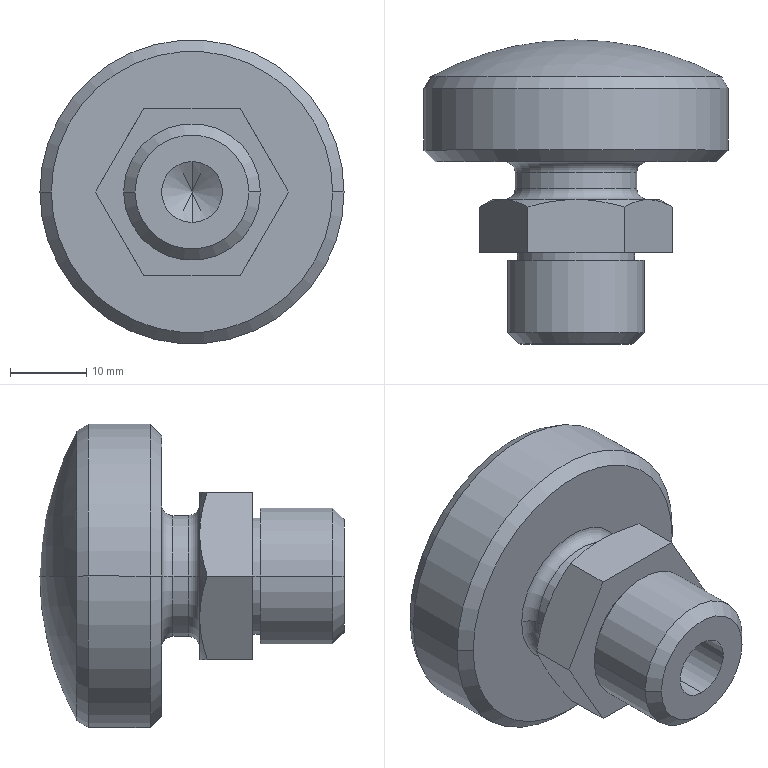Component | SolidWorks | BreatherCap-1 | 1 solid | 37 faces | box 40 x 40 x 40 mm | volume 21828 mm3 | plane 11 | cylinder 10 | cone 10 | torus 4 | sphere 2 | commonest cylinder face diameters 8 x2 15.4 x2 18 x2 16 x2 39.997 x2 | material Q235-A
STEP:
#1=COLOUR_RGB('',0.7922,0.8196,0.9333);
#2=FILL_AREA_STYLE_COLOUR('',#1);
#3=FILL_AREA_STYLE('',(#2));
#4=SURFACE_STYLE_FILL_AREA(#3);
#5=SURFACE_SIDE_STYLE('',(#4));
#6=SURFACE_STYLE_USAGE(.BOTH.,#5);
#7=PRESENTATION_STYLE_ASSIGNMENT((#6));
#8=CARTESIAN_POINT('',(-14.961,3.78,0.1575));
#9=VERTEX_POINT('',#8);
#10=CARTESIAN_POINT('',(-14.961,3.78,-0.1575));
#11=VERTEX_POINT('',#10);
#12=CARTESIAN_POINT('',(-14.961,3.78,0.));
#13=DIRECTION('',(0.,-1.,0.));
#14=DIRECTION('',(0.,0.,-1.));
#15=AXIS2_PLACEMENT_3D('',#12,#13,#14);
#16=CIRCLE('',#15,0.1575);
#17=EDGE_CURVE('',#9,#11,#16,.T.);
#18=ORIENTED_EDGE('',*,*,#17,.F.);
#19=CARTESIAN_POINT('',(-14.961,2.48,0.1575));
#20=VERTEX_POINT('',#19);
#21=CARTESIAN_POINT('',(-14.961,2.48,0.1575));
#22=DIRECTION('',(0.,-1.,0.));
#23=VECTOR('',#22,39.37);
#24=LINE('',#21,#23);
#25=EDGE_CURVE('',#9,#20,#24,.T.);
#26=ORIENTED_EDGE('',*,*,#25,.T.);
#27=CARTESIAN_POINT('',(-14.961,2.48,-0.1575));
#28=VERTEX_POINT('',#27);
#29=CARTESIAN_POINT('',(-14.961,2.48,0.));
#30=DIRECTION('',(0.,-1.,0.));
#31=DIRECTION('',(0.,0.,-1.));
#32=AXIS2_PLACEMENT_3D('',#29,#30,#31);
#33=CIRCLE('',#32,0.1575);
#34=EDGE_CURVE('',#20,#28,#33,.T.);
#35=ORIENTED_EDGE('',*,*,#34,.T.);
#36=CARTESIAN_POINT('',(-14.961,2.48,-0.1575));
#37=DIRECTION('',(0.,-1.,0.));
#38=VECTOR('',#37,39.37);
#39=LINE('',#36,#38);
#40=EDGE_CURVE('',#11,#28,#39,.T.);
#41=ORIENTED_EDGE('',*,*,#40,.F.);
#42=EDGE_LOOP('',(#18,#26,#35,#41));
#43=FACE_OUTER_BOUND('',#42,.T.);
#44=CARTESIAN_POINT('',(-14.961,2.48,0.));
#45=DIRECTION('',(0.,-1.,0.));
#46=DIRECTION('',(0.,0.,-1.));
#47=AXIS2_PLACEMENT_3D('',#44,#45,#46);
#48=CYLINDRICAL_SURFACE('',#47,0.1575);
#49=ADVANCED_FACE('',(#43),#48,.F.);
#50=CARTESIAN_POINT('',(-14.961,3.874,0.));
#51=VERTEX_POINT('',#50);
#52=CARTESIAN_POINT('',(-14.961,3.78,-0.1575));
#53=DIRECTION('',(0.,-0.515,-0.8572));
#54=VECTOR('',#53,39.37);
#55=LINE('',#52,#54);
#56=EDGE_CURVE('',#51,#11,#55,.T.);
#57=ORIENTED_EDGE('',*,*,#56,.F.);
#58=CARTESIAN_POINT('',(-14.961,3.78,0.1575));
#59=DIRECTION('',(0.,-0.515,0.8572));
#60=VECTOR('',#59,39.37);
#61=LINE('',#58,#60);
#62=EDGE_CURVE('',#51,#9,#61,.T.);
#63=ORIENTED_EDGE('',*,*,#62,.T.);
#64=ORIENTED_EDGE('',*,*,#17,.T.);
#65=EDGE_LOOP('',(#57,#63,#64));
#66=FACE_OUTER_BOUND('',#65,.T.);
#67=CARTESIAN_POINT('',(-14.961,3.78,0.));
#68=DIRECTION('',(0.,-1.,0.));
#69=DIRECTION('',(0.,0.,-1.));
#70=AXIS2_PLACEMENT_3D('',#67,#68,#69);
#71=CONICAL_SURFACE('',#70,0.1575,1.03);
#72=ADVANCED_FACE('',(#66),#71,.F.);
#73=CARTESIAN_POINT('',(-15.264,2.913,0.));
#74=VERTEX_POINT('',#73);
#75=CARTESIAN_POINT('',(-14.657,2.913,0.));
#76=VERTEX_POINT('',#75);
#77=CARTESIAN_POINT('',(-14.961,2.913,0.));
#78=DIRECTION('',(-0.,1.,0.));
#79=DIRECTION('',(-1.,-0.,0.));
#80=AXIS2_PLACEMENT_3D('',#77,#78,#79);
#81=CIRCLE('',#80,0.3031);
#82=EDGE_CURVE('',#74,#76,#81,.T.);
#83=ORIENTED_EDGE('',*,*,#82,.T.);
#84=CARTESIAN_POINT('',(-14.657,2.953,0.));
#85=VERTEX_POINT('',#84);
#86=CARTESIAN_POINT('',(-14.657,4.055,0.));
#87=DIRECTION('',(-0.,1.,0.));
#88=VECTOR('',#87,39.37);
#89=LINE('',#86,#88);
#90=EDGE_CURVE('',#76,#85,#89,.T.);
#91=ORIENTED_EDGE('',*,*,#90,.T.);
#92=CARTESIAN_POINT('',(-15.264,2.953,0.));
#93=VERTEX_POINT('',#92);
#94=CARTESIAN_POINT('',(-14.961,2.953,0.));
#95=DIRECTION('',(-0.,1.,0.));
#96=DIRECTION('',(-1.,-0.,0.));
#97=AXIS2_PLACEMENT_3D('',#94,#95,#96);
#98=CIRCLE('',#97,0.3031);
#99=EDGE_CURVE('',#93,#85,#98,.T.);
#100=ORIENTED_EDGE('',*,*,#99,.F.);
#101=CARTESIAN_POINT('',(-15.264,4.055,0.));
#102=DIRECTION('',(-0.,1.,0.));
#103=VECTOR('',#102,39.37);
#104=LINE('',#101,#103);
#105=EDGE_CURVE('',#74,#93,#104,.T.);
#106=ORIENTED_EDGE('',*,*,#105,.F.);
#107=EDGE_LOOP('',(#83,#91,#100,#106));
#108=FACE_OUTER_BOUND('',#107,.T.);
#109=CARTESIAN_POINT('',(-14.961,4.055,0.));
#110=DIRECTION('',(-0.,1.,0.));
#111=DIRECTION('',(-1.,-0.,0.));
#112=AXIS2_PLACEMENT_3D('',#109,#110,#111);
#113=CYLINDRICAL_SURFACE('',#112,0.3031);
#114=ADVANCED_FACE('',(#108),#113,.T.);
#115=CARTESIAN_POINT('',(-15.315,2.539,0.));
#116=VERTEX_POINT('',#115);
#117=CARTESIAN_POINT('',(-14.606,2.539,0.));
#118=VERTEX_POINT('',#117);
#119=CARTESIAN_POINT('',(-14.961,2.539,0.));
#120=DIRECTION('',(-0.,1.,0.));
#121=DIRECTION('',(-1.,-0.,0.));
#122=AXIS2_PLACEMENT_3D('',#119,#120,#121);
#123=CIRCLE('',#122,0.3543);
#124=EDGE_CURVE('',#116,#118,#123,.T.);
#125=ORIENTED_EDGE('',*,*,#124,.T.);
#126=CARTESIAN_POINT('',(-14.606,2.913,0.));
#127=VERTEX_POINT('',#126);
#128=CARTESIAN_POINT('',(-14.606,4.055,0.));
#129=DIRECTION('',(-0.,1.,0.));
#130=VECTOR('',#129,39.37);
#131=LINE('',#128,#130);
#132=EDGE_CURVE('',#118,#127,#131,.T.);
#133=ORIENTED_EDGE('',*,*,#132,.T.);
#134=CARTESIAN_POINT('',(-15.315,2.913,0.));
#135=VERTEX_POINT('',#134);
#136=CARTESIAN_POINT('',(-14.961,2.913,0.));
#137=DIRECTION('',(-0.,1.,0.));
#138=DIRECTION('',(-1.,-0.,0.));
#139=AXIS2_PLACEMENT_3D('',#136,#137,#138);
#140=CIRCLE('',#139,0.3543);
#141=EDGE_CURVE('',#135,#127,#140,.T.);
#142=ORIENTED_EDGE('',*,*,#141,.F.);
#143=CARTESIAN_POINT('',(-15.315,4.055,0.));
#144=DIRECTION('',(-0.,1.,0.));
#145=VECTOR('',#144,39.37);
#146=LINE('',#143,#145);
#147=EDGE_CURVE('',#116,#135,#146,.T.);
#148=ORIENTED_EDGE('',*,*,#147,.F.);
#149=EDGE_LOOP('',(#125,#133,#142,#148));
#150=FACE_OUTER_BOUND('',#149,.T.);
#151=CARTESIAN_POINT('',(-14.961,4.055,0.));
#152=DIRECTION('',(-0.,1.,0.));
#153=DIRECTION('',(-1.,-0.,0.));
#154=AXIS2_PLACEMENT_3D('',#151,#152,#153);
#155=CYLINDRICAL_SURFACE('',#154,0.3543);
#156=ADVANCED_FACE('',(#150),#155,.T.);
#157=CARTESIAN_POINT('',(-15.256,2.48,0.));
#158=VERTEX_POINT('',#157);
#159=CARTESIAN_POINT('',(-14.665,2.48,0.));
#160=VERTEX_POINT('',#159);
#161=CARTESIAN_POINT('',(-14.961,2.48,0.));
#162=DIRECTION('',(-0.,1.,0.));
#163=DIRECTION('',(-1.,-0.,0.));
#164=AXIS2_PLACEMENT_3D('',#161,#162,#163);
#165=CIRCLE('',#164,0.2953);
#166=EDGE_CURVE('',#158,#160,#165,.T.);
#167=ORIENTED_EDGE('',*,*,#166,.T.);
#168=CARTESIAN_POINT('',(-14.665,2.48,0.));
#169=DIRECTION('',(0.7071,0.7071,0.));
#170=VECTOR('',#169,39.37);
#171=LINE('',#168,#170);
#172=EDGE_CURVE('',#160,#118,#171,.T.);
#173=ORIENTED_EDGE('',*,*,#172,.T.);
#174=ORIENTED_EDGE('',*,*,#124,.F.);
#175=CARTESIAN_POINT('',(-15.256,2.48,0.));
#176=DIRECTION('',(-0.7071,0.7071,0.));
#177=VECTOR('',#176,39.37);
#178=LINE('',#175,#177);
#179=EDGE_CURVE('',#158,#116,#178,.T.);
#180=ORIENTED_EDGE('',*,*,#179,.F.);
#181=EDGE_LOOP('',(#167,#173,#174,#180));
#182=FACE_OUTER_BOUND('',#181,.T.);
#183=CARTESIAN_POINT('',(-14.961,2.48,0.));
#184=DIRECTION('',(-0.,1.,0.));
#185=DIRECTION('',(-1.,-0.,0.));
#186=AXIS2_PLACEMENT_3D('',#183,#184,#185);
#187=CONICAL_SURFACE('',#186,0.2953,0.7854);
#188=ADVANCED_FACE('',(#182),#187,.T.);
#189=CARTESIAN_POINT('',(-14.961,3.228,-0.4318));
#190=VERTEX_POINT('',#189);
#191=CARTESIAN_POINT('',(-14.961,3.228,0.4318));
#192=VERTEX_POINT('',#191);
#193=CARTESIAN_POINT('',(-14.961,3.228,0.));
#194=DIRECTION('',(0.,-1.,0.));
#195=DIRECTION('',(0.,0.,-1.));
#196=AXIS2_PLACEMENT_3D('',#193,#194,#195);
#197=CIRCLE('',#196,0.4318);
#198=EDGE_CURVE('',#190,#192,#197,.T.);
#199=ORIENTED_EDGE('',*,*,#198,.T.);
#200=CARTESIAN_POINT('',(-14.961,3.228,0.433));
#201=VERTEX_POINT('',#200);
#202=CARTESIAN_POINT('',(-14.961,3.228,0.4318));
#203=DIRECTION('',(0.,-0.5,0.866));
#204=VECTOR('',#203,39.37);
#205=LINE('',#202,#204);
#206=EDGE_CURVE('',#192,#201,#205,.T.);
#207=ORIENTED_EDGE('',*,*,#206,.T.);
#208=CARTESIAN_POINT('',(-14.711,3.189,0.433));
#209=VERTEX_POINT('',#208);
#210=CARTESIAN_POINT('',(-14.961,3.228,0.433));
#211=CARTESIAN_POINT('',(-14.939,3.228,0.433));
#212=CARTESIAN_POINT('',(-14.918,3.227,0.433));
#213=CARTESIAN_POINT('',(-14.876,3.223,0.433));
#214=CARTESIAN_POINT('',(-14.855,3.221,0.433));
#215=CARTESIAN_POINT('',(-14.792,3.21,0.433));
#216=CARTESIAN_POINT('',(-14.751,3.201,0.433));
#217=CARTESIAN_POINT('',(-14.711,3.189,0.433));
#218=B_SPLINE_CURVE_WITH_KNOTS('',3,(#210,#211,#212,#213,#214,#215,#216,#217),.UNSPECIFIED.,.F.,.F.,(4,2,2,4),(0.01775,0.01936,0.02096,0.02418),.UNSPECIFIED.);
#219=EDGE_CURVE('',#201,#209,#218,.T.);
#220=ORIENTED_EDGE('',*,*,#219,.T.);
#221=CARTESIAN_POINT('',(-14.461,3.189,0.));
#222=VERTEX_POINT('',#221);
#223=CARTESIAN_POINT('',(-14.711,3.189,0.433));
#224=CARTESIAN_POINT('',(-14.69,3.201,0.3977));
#225=CARTESIAN_POINT('',(-14.67,3.21,0.3621));
#226=CARTESIAN_POINT('',(-14.628,3.224,0.2901));
#227=CARTESIAN_POINT('',(-14.607,3.228,0.2537));
#228=CARTESIAN_POINT('',(-14.575,3.228,0.1985));
#229=CARTESIAN_POINT('',(-14.565,3.227,0.18));
#230=CARTESIAN_POINT('',(-14.543,3.223,0.1434));
#231=CARTESIAN_POINT('',(-14.533,3.221,0.1253));
#232=CARTESIAN_POINT('',(-14.502,3.211,0.07109));
#233=CARTESIAN_POINT('',(-14.481,3.201,0.0354));
#234=CARTESIAN_POINT('',(-14.461,3.189,0.));
#235=B_SPLINE_CURVE_WITH_KNOTS('',3,(#223,#224,#225,#226,#227,#228,#229,#230,#231,#232,#233,#234),.UNSPECIFIED.,.F.,.F.,(4,2,2,2,2,4),(0.00000024,0.003207,0.006413,0.008017,0.00962,0.01283),.UNSPECIFIED.);
#236=EDGE_CURVE('',#209,#222,#235,.T.);
#237=ORIENTED_EDGE('',*,*,#236,.T.);
#238=CARTESIAN_POINT('',(-14.711,3.189,-0.433));
#239=VERTEX_POINT('',#238);
#240=CARTESIAN_POINT('',(-14.461,3.189,0.));
#241=CARTESIAN_POINT('',(-14.481,3.201,-0.03535));
#242=CARTESIAN_POINT('',(-14.502,3.21,-0.07096));
#243=CARTESIAN_POINT('',(-14.543,3.224,-0.1429));
#244=CARTESIAN_POINT('',(-14.564,3.228,-0.1793));
#245=CARTESIAN_POINT('',(-14.596,3.228,-0.2345));
#246=CARTESIAN_POINT('',(-14.607,3.227,-0.253));
#247=CARTESIAN_POINT('',(-14.628,3.223,-0.2896));
#248=CARTESIAN_POINT('',(-14.638,3.221,-0.3077));
#249=CARTESIAN_POINT('',(-14.67,3.211,-0.3619));
#250=CARTESIAN_POINT('',(-14.69,3.201,-0.3976));
#251=CARTESIAN_POINT('',(-14.711,3.189,-0.433));
#252=B_SPLINE_CURVE_WITH_KNOTS('',3,(#240,#241,#242,#243,#244,#245,#246,#247,#248,#249,#250,#251),.UNSPECIFIED.,.F.,.F.,(4,2,2,2,2,4),(0.00000024,0.003207,0.006413,0.008017,0.00962,0.01283),.UNSPECIFIED.);
#253=EDGE_CURVE('',#222,#239,#252,.T.);
#254=ORIENTED_EDGE('',*,*,#253,.T.);
#255=CARTESIAN_POINT('',(-14.961,3.228,-0.433));
#256=VERTEX_POINT('',#255);
#257=CARTESIAN_POINT('',(-14.711,3.189,-0.433));
#258=CARTESIAN_POINT('',(-14.751,3.201,-0.433));
#259=CARTESIAN_POINT('',(-14.792,3.21,-0.433));
#260=CARTESIAN_POINT('',(-14.855,3.221,-0.433));
#261=CARTESIAN_POINT('',(-14.876,3.223,-0.433));
#262=CARTESIAN_POINT('',(-14.918,3.227,-0.433));
#263=CARTESIAN_POINT('',(-14.939,3.228,-0.433));
#264=CARTESIAN_POINT('',(-14.961,3.228,-0.433));
#265=B_SPLINE_CURVE_WITH_KNOTS('',3,(#257,#258,#259,#260,#261,#262,#263,#264),.UNSPECIFIED.,.F.,.F.,(4,2,2,4),(0.004658,0.007863,0.009466,0.01107),.UNSPECIFIED.);
#266=EDGE_CURVE('',#239,#256,#265,.T.);
#267=ORIENTED_EDGE('',*,*,#266,.T.);
#268=CARTESIAN_POINT('',(-14.961,3.228,-0.4318));
#269=DIRECTION('',(0.,-0.5,-0.866));
#270=VECTOR('',#269,39.37);
#271=LINE('',#268,#270);
#272=EDGE_CURVE('',#190,#256,#271,.T.);
#273=ORIENTED_EDGE('',*,*,#272,.F.);
#274=EDGE_LOOP('',(#199,#207,#220,#237,#254,#267,#273));
#275=FACE_OUTER_BOUND('',#274,.T.);
#276=CARTESIAN_POINT('',(-14.961,3.228,0.));
#277=DIRECTION('',(0.,-1.,0.));
#278=DIRECTION('',(0.,0.,-1.));
#279=AXIS2_PLACEMENT_3D('',#276,#277,#278);
#280=CONICAL_SURFACE('',#279,0.4318,1.047);
#281=ADVANCED_FACE('',(#275),#280,.T.);
#282=CARTESIAN_POINT('',(-14.646,3.287,0.));
#283=VERTEX_POINT('',#282);
#284=CARTESIAN_POINT('',(-15.276,3.287,0.));
#285=VERTEX_POINT('',#284);
#286=CARTESIAN_POINT('',(-14.961,3.287,0.));
#287=DIRECTION('',(-0.,1.,0.));
#288=DIRECTION('',(-1.,-0.,0.));
#289=AXIS2_PLACEMENT_3D('',#286,#287,#288);
#290=CIRCLE('',#289,0.315);
#291=EDGE_CURVE('',#283,#285,#290,.T.);
#292=ORIENTED_EDGE('',*,*,#291,.F.);
#293=CARTESIAN_POINT('',(-14.587,3.228,0.));
#294=VERTEX_POINT('',#293);
#295=CARTESIAN_POINT('',(-14.587,3.287,0.));
#296=DIRECTION('',(-0.,-0.,1.));
#297=DIRECTION('',(1.,0.,0.));
#298=AXIS2_PLACEMENT_3D('',#295,#296,#297);
#299=CIRCLE('',#298,0.05906);
#300=EDGE_CURVE('',#283,#294,#299,.T.);
#301=ORIENTED_EDGE('',*,*,#300,.T.);
#302=CARTESIAN_POINT('',(-15.335,3.228,0.));
#303=VERTEX_POINT('',#302);
#304=CARTESIAN_POINT('',(-14.961,3.228,0.));
#305=DIRECTION('',(-0.,1.,0.));
#306=DIRECTION('',(-1.,-0.,0.));
#307=AXIS2_PLACEMENT_3D('',#304,#305,#306);
#308=CIRCLE('',#307,0.374);
#309=EDGE_CURVE('',#294,#303,#308,.T.);
#310=ORIENTED_EDGE('',*,*,#309,.T.);
#311=CARTESIAN_POINT('',(-15.335,3.287,0.));
#312=DIRECTION('',(0.,0.,-1.));
#313=DIRECTION('',(-1.,0.,0.));
#314=AXIS2_PLACEMENT_3D('',#311,#312,#313);
#315=CIRCLE('',#314,0.05906);
#316=EDGE_CURVE('',#285,#303,#315,.T.);
#317=ORIENTED_EDGE('',*,*,#316,.F.);
#318=EDGE_LOOP('',(#292,#301,#310,#317));
#319=FACE_OUTER_BOUND('',#318,.T.);
#320=CARTESIAN_POINT('',(-14.961,3.287,0.));
#321=DIRECTION('',(-0.,1.,0.));
#322=DIRECTION('',(-1.,-0.,0.));
#323=AXIS2_PLACEMENT_3D('',#320,#321,#322);
#324=TOROIDAL_SURFACE('',#323,0.374,0.05906);
#325=ADVANCED_FACE('',(#319),#324,.F.);
#326=CARTESIAN_POINT('',(-14.961,3.287,0.));
#327=DIRECTION('',(-0.,1.,0.));
#328=DIRECTION('',(-1.,-0.,0.));
#329=AXIS2_PLACEMENT_3D('',#326,#327,#328);
#330=CIRCLE('',#329,0.315);
#331=EDGE_CURVE('',#285,#283,#330,.T.);
#332=ORIENTED_EDGE('',*,*,#331,.T.);
#333=CARTESIAN_POINT('',(-14.646,3.366,0.));
#334=VERTEX_POINT('',#333);
#335=CARTESIAN_POINT('',(-14.646,4.055,0.));
#336=DIRECTION('',(-0.,1.,0.));
#337=VECTOR('',#336,39.37);
#338=LINE('',#335,#337);
#339=EDGE_CURVE('',#283,#334,#338,.T.);
#340=ORIENTED_EDGE('',*,*,#339,.T.);
#341=CARTESIAN_POINT('',(-15.276,3.366,0.));
#342=VERTEX_POINT('',#341);
#343=CARTESIAN_POINT('',(-14.961,3.366,0.));
#344=DIRECTION('',(-0.,1.,0.));
#345=DIRECTION('',(-1.,-0.,0.));
#346=AXIS2_PLACEMENT_3D('',#343,#344,#345);
#347=CIRCLE('',#346,0.315);
#348=EDGE_CURVE('',#342,#334,#347,.T.);
#349=ORIENTED_EDGE('',*,*,#348,.F.);
#350=CARTESIAN_POINT('',(-15.276,4.055,0.));
#351=DIRECTION('',(-0.,1.,0.));
#352=VECTOR('',#351,39.37);
#353=LINE('',#350,#352);
#354=EDGE_CURVE('',#285,#342,#353,.T.);
#355=ORIENTED_EDGE('',*,*,#354,.F.);
#356=EDGE_LOOP('',(#332,#340,#349,#355));
#357=FACE_OUTER_BOUND('',#356,.T.);
#358=CARTESIAN_POINT('',(-14.961,4.055,0.));
#359=DIRECTION('',(-0.,1.,0.));
#360=DIRECTION('',(-1.,-0.,0.));
#361=AXIS2_PLACEMENT_3D('',#358,#359,#360);
#362=CYLINDRICAL_SURFACE('',#361,0.315);
#363=ADVANCED_FACE('',(#357),#362,.T.);
#364=CARTESIAN_POINT('',(-14.587,3.425,0.));
#365=VERTEX_POINT('',#364);
#366=CARTESIAN_POINT('',(-15.335,3.425,0.));
#367=VERTEX_POINT('',#366);
#368=CARTESIAN_POINT('',(-14.961,3.425,0.));
#369=DIRECTION('',(-0.,1.,0.));
#370=DIRECTION('',(-1.,-0.,0.));
#371=AXIS2_PLACEMENT_3D('',#368,#369,#370);
#372=CIRCLE('',#371,0.374);
#373=EDGE_CURVE('',#365,#367,#372,.T.);
#374=ORIENTED_EDGE('',*,*,#373,.F.);
#375=CARTESIAN_POINT('',(-14.587,3.366,0.));
#376=DIRECTION('',(-0.,-0.,1.));
#377=DIRECTION('',(1.,0.,0.));
#378=AXIS2_PLACEMENT_3D('',#375,#376,#377);
#379=CIRCLE('',#378,0.05906);
#380=EDGE_CURVE('',#365,#334,#379,.T.);
#381=ORIENTED_EDGE('',*,*,#380,.T.);
#382=CARTESIAN_POINT('',(-14.961,3.366,0.));
#383=DIRECTION('',(-0.,1.,0.));
#384=DIRECTION('',(-1.,-0.,0.));
#385=AXIS2_PLACEMENT_3D('',#382,#383,#384);
#386=CIRCLE('',#385,0.315);
#387=EDGE_CURVE('',#334,#342,#386,.T.);
#388=ORIENTED_EDGE('',*,*,#387,.T.);
#389=CARTESIAN_POINT('',(-15.335,3.366,0.));
#390=DIRECTION('',(0.,0.,-1.));
#391=DIRECTION('',(-1.,0.,0.));
#392=AXIS2_PLACEMENT_3D('',#389,#390,#391);
#393=CIRCLE('',#392,0.05906);
#394=EDGE_CURVE('',#367,#342,#393,.T.);
#395=ORIENTED_EDGE('',*,*,#394,.F.);
#396=EDGE_LOOP('',(#374,#381,#388,#395));
#397=FACE_OUTER_BOUND('',#396,.T.);
#398=CARTESIAN_POINT('',(-14.961,3.366,0.));
#399=DIRECTION('',(-0.,1.,0.));
#400=DIRECTION('',(-1.,-0.,0.));
#401=AXIS2_PLACEMENT_3D('',#398,#399,#400);
#402=TOROIDAL_SURFACE('',#401,0.374,0.05906);
#403=ADVANCED_FACE('',(#397),#402,.F.);
#404=CARTESIAN_POINT('',(-15.689,3.425,0.));
#405=VERTEX_POINT('',#404);
#406=CARTESIAN_POINT('',(-14.232,3.425,0.));
#407=VERTEX_POINT('',#406);
#408=CARTESIAN_POINT('',(-14.961,3.425,0.));
#409=DIRECTION('',(-0.,1.,0.));
#410=DIRECTION('',(-1.,-0.,0.));
#411=AXIS2_PLACEMENT_3D('',#408,#409,#410);
#412=CIRCLE('',#411,0.7283);
#413=EDGE_CURVE('',#405,#407,#412,.T.);
#414=ORIENTED_EDGE('',*,*,#413,.T.);
#415=CARTESIAN_POINT('',(-14.173,3.484,0.));
#416=VERTEX_POINT('',#415);
#417=CARTESIAN_POINT('',(-14.232,3.425,0.));
#418=DIRECTION('',(0.7071,0.7071,0.));
#419=VECTOR('',#418,39.37);
#420=LINE('',#417,#419);
#421=EDGE_CURVE('',#407,#416,#420,.T.);
#422=ORIENTED_EDGE('',*,*,#421,.T.);
#423=CARTESIAN_POINT('',(-15.748,3.484,0.));
#424=VERTEX_POINT('',#423);
#425=CARTESIAN_POINT('',(-14.961,3.484,0.));
#426=DIRECTION('',(-0.,1.,0.));
#427=DIRECTION('',(-1.,-0.,0.));
#428=AXIS2_PLACEMENT_3D('',#425,#426,#427);
#429=CIRCLE('',#428,0.7873);
#430=EDGE_CURVE('',#424,#416,#429,.T.);
#431=ORIENTED_EDGE('',*,*,#430,.F.);
#432=CARTESIAN_POINT('',(-15.689,3.425,0.));
#433=DIRECTION('',(-0.7071,0.7071,0.));
#434=VECTOR('',#433,39.37);
#435=LINE('',#432,#434);
#436=EDGE_CURVE('',#405,#424,#435,.T.);
#437=ORIENTED_EDGE('',*,*,#436,.F.);
#438=EDGE_LOOP('',(#414,#422,#431,#437));
#439=FACE_OUTER_BOUND('',#438,.T.);
#440=CARTESIAN_POINT('',(-14.961,3.425,0.));
#441=DIRECTION('',(-0.,1.,0.));
#442=DIRECTION('',(-1.,-0.,0.));
#443=AXIS2_PLACEMENT_3D('',#440,#441,#442);
#444=CONICAL_SURFACE('',#443,0.7283,0.7854);
#445=ADVANCED_FACE('',(#439),#444,.T.);
#446=ORIENTED_EDGE('',*,*,#430,.T.);
#447=CARTESIAN_POINT('',(-14.173,3.804,0.));
#448=VERTEX_POINT('',#447);
#449=CARTESIAN_POINT('',(-14.173,4.055,0.));
#450=DIRECTION('',(-0.,1.,0.));
#451=VECTOR('',#450,39.37);
#452=LINE('',#449,#451);
#453=EDGE_CURVE('',#416,#448,#452,.T.);
#454=ORIENTED_EDGE('',*,*,#453,.T.);
#455=CARTESIAN_POINT('',(-15.748,3.804,0.));
#456=VERTEX_POINT('',#455);
#457=CARTESIAN_POINT('',(-14.961,3.804,0.));
#458=DIRECTION('',(-0.,1.,0.));
#459=DIRECTION('',(-1.,-0.,0.));
#460=AXIS2_PLACEMENT_3D('',#457,#458,#459);
#461=CIRCLE('',#460,0.7873);
#462=EDGE_CURVE('',#456,#448,#461,.T.);
#463=ORIENTED_EDGE('',*,*,#462,.F.);
#464=CARTESIAN_POINT('',(-15.748,4.055,0.));
#465=DIRECTION('',(-0.,1.,0.));
#466=VECTOR('',#465,39.37);
#467=LINE('',#464,#466);
#468=EDGE_CURVE('',#424,#456,#467,.T.);
#469=ORIENTED_EDGE('',*,*,#468,.F.);
#470=EDGE_LOOP('',(#446,#454,#463,#469));
#471=FACE_OUTER_BOUND('',#470,.T.);
#472=CARTESIAN_POINT('',(-14.961,4.055,0.));
#473=DIRECTION('',(-0.,1.,0.));
#474=DIRECTION('',(-1.,-0.,0.));
#475=AXIS2_PLACEMENT_3D('',#472,#473,#474);
#476=CYLINDRICAL_SURFACE('',#475,0.7873);
#477=ADVANCED_FACE('',(#471),#476,.T.);
#478=CARTESIAN_POINT('',(-15.714,3.863,0.));
#479=VERTEX_POINT('',#478);
#480=CARTESIAN_POINT('',(-14.207,3.863,0.));
#481=VERTEX_POINT('',#480);
#482=CARTESIAN_POINT('',(-14.961,3.863,0.));
#483=DIRECTION('',(-0.,1.,0.));
#484=DIRECTION('',(-1.,-0.,0.));
#485=AXIS2_PLACEMENT_3D('',#482,#483,#484);
#486=CIRCLE('',#485,0.7532);
#487=EDGE_CURVE('',#479,#481,#486,.T.);
#488=ORIENTED_EDGE('',*,*,#487,.F.);
#489=CARTESIAN_POINT('',(-15.748,3.804,0.));
#490=DIRECTION('',(-0.5,-0.866,0.));
#491=VECTOR('',#490,39.37);
#492=LINE('',#489,#491);
#493=EDGE_CURVE('',#479,#456,#492,.T.);
#494=ORIENTED_EDGE('',*,*,#493,.T.);
#495=ORIENTED_EDGE('',*,*,#462,.T.);
#496=CARTESIAN_POINT('',(-14.173,3.804,0.));
#497=DIRECTION('',(0.5,-0.866,0.));
#498=VECTOR('',#497,39.37);
#499=LINE('',#496,#498);
#500=EDGE_CURVE('',#481,#448,#499,.T.);
#501=ORIENTED_EDGE('',*,*,#500,.F.);
#502=EDGE_LOOP('',(#488,#494,#495,#501));
#503=FACE_OUTER_BOUND('',#502,.T.);
#504=CARTESIAN_POINT('',(-14.961,3.804,0.));
#505=DIRECTION('',(0.,-1.,0.));
#506=DIRECTION('',(1.,0.,0.));
#507=AXIS2_PLACEMENT_3D('',#504,#505,#506);
#508=CONICAL_SURFACE('',#507,0.7873,0.5236);
#509=ADVANCED_FACE('',(#503),#508,.T.);
#510=CARTESIAN_POINT('',(-14.961,3.863,0.));
#511=DIRECTION('',(-0.,1.,0.));
#512=DIRECTION('',(-1.,-0.,0.));
#513=AXIS2_PLACEMENT_3D('',#510,#511,#512);
#514=CIRCLE('',#513,0.7532);
#515=EDGE_CURVE('',#481,#479,#514,.T.);
#516=ORIENTED_EDGE('',*,*,#515,.T.);
#517=CARTESIAN_POINT('',(-14.961,4.055,0.));
#518=VERTEX_POINT('',#517);
#519=CARTESIAN_POINT('',(-14.961,2.48,0.));
#520=DIRECTION('',(0.,0.,-1.));
#521=DIRECTION('',(-1.,0.,-0.));
#522=AXIS2_PLACEMENT_3D('',#519,#520,#521);
#523=CIRCLE('',#522,1.575);
#524=EDGE_CURVE('',#479,#518,#523,.T.);
#525=ORIENTED_EDGE('',*,*,#524,.T.);
#526=CARTESIAN_POINT('',(-14.961,2.48,0.));
#527=DIRECTION('',(0.,0.,1.));
#528=DIRECTION('',(1.,0.,0.));
#529=AXIS2_PLACEMENT_3D('',#526,#527,#528);
#530=CIRCLE('',#529,1.575);
#531=EDGE_CURVE('',#481,#518,#530,.T.);
#532=ORIENTED_EDGE('',*,*,#531,.F.);
#533=EDGE_LOOP('',(#516,#525,#532));
#534=FACE_OUTER_BOUND('',#533,.T.);
#535=CARTESIAN_POINT('',(-14.961,2.48,0.));
#536=DIRECTION('',(0.,0.,-1.));
#537=DIRECTION('',(1.,0.,0.));
#538=AXIS2_PLACEMENT_3D('',#535,#536,#537);
#539=SPHERICAL_SURFACE('',#538,1.575);
#540=ADVANCED_FACE('',(#534),#539,.T.);
#541=CARTESIAN_POINT('',(-14.961,3.228,0.));
#542=DIRECTION('',(-0.,1.,0.));
#543=DIRECTION('',(-1.,-0.,0.));
#544=AXIS2_PLACEMENT_3D('',#541,#542,#543);
#545=CIRCLE('',#544,0.374);
#546=EDGE_CURVE('',#303,#294,#545,.T.);
#547=ORIENTED_EDGE('',*,*,#546,.F.);
#548=ORIENTED_EDGE('',*,*,#309,.F.);
#549=EDGE_LOOP('',(#547,#548));
#550=FACE_BOUND('',#549,.T.);
#551=ORIENTED_EDGE('',*,*,#198,.F.);
#552=CARTESIAN_POINT('',(-14.961,3.228,0.));
#553=DIRECTION('',(0.,-1.,0.));
#554=DIRECTION('',(0.,0.,-1.));
#555=AXIS2_PLACEMENT_3D('',#552,#553,#554);
#556=CIRCLE('',#555,0.4318);
#557=EDGE_CURVE('',#192,#190,#556,.T.);
#558=ORIENTED_EDGE('',*,*,#557,.F.);
#559=EDGE_LOOP('',(#551,#558));
#560=FACE_OUTER_BOUND('',#559,.T.);
#561=CARTESIAN_POINT('',(-14.461,3.228,0.));
#562=DIRECTION('',(0.,-1.,0.));
#563=DIRECTION('',(1.,0.,0.));
#564=AXIS2_PLACEMENT_3D('',#561,#562,#563);
#565=PLANE('',#564);
#566=ADVANCED_FACE('',(#550,#560),#565,.F.);
#567=ORIENTED_EDGE('',*,*,#524,.F.);
#568=ORIENTED_EDGE('',*,*,#487,.T.);
#569=ORIENTED_EDGE('',*,*,#531,.T.);
#570=EDGE_LOOP('',(#567,#568,#569));
#571=FACE_OUTER_BOUND('',#570,.T.);
#572=CARTESIAN_POINT('',(-14.961,2.48,0.));
#573=DIRECTION('',(0.,0.,-1.));
#574=DIRECTION('',(1.,0.,0.));
#575=AXIS2_PLACEMENT_3D('',#572,#573,#574);
#576=SPHERICAL_SURFACE('',#575,1.575);
#577=ADVANCED_FACE('',(#571),#576,.T.);
#578=ORIENTED_EDGE('',*,*,#493,.F.);
#579=ORIENTED_EDGE('',*,*,#515,.F.);
#580=ORIENTED_EDGE('',*,*,#500,.T.);
#581=CARTESIAN_POINT('',(-14.961,3.804,0.));
#582=DIRECTION('',(-0.,1.,0.));
#583=DIRECTION('',(-1.,-0.,0.));
#584=AXIS2_PLACEMENT_3D('',#581,#582,#583);
#585=CIRCLE('',#584,0.7873);
#586=EDGE_CURVE('',#448,#456,#585,.T.);
#587=ORIENTED_EDGE('',*,*,#586,.T.);
#588=EDGE_LOOP('',(#578,#579,#580,#587));
#589=FACE_OUTER_BOUND('',#588,.T.);
#590=CARTESIAN_POINT('',(-14.961,3.804,0.));
#591=DIRECTION('',(0.,-1.,0.));
#592=DIRECTION('',(1.,0.,0.));
#593=AXIS2_PLACEMENT_3D('',#590,#591,#592);
#594=CONICAL_SURFACE('',#593,0.7873,0.5236);
#595=ADVANCED_FACE('',(#589),#594,.T.);
#596=ORIENTED_EDGE('',*,*,#453,.F.);
#597=CARTESIAN_POINT('',(-14.961,3.484,0.));
#598=DIRECTION('',(-0.,1.,0.));
#599=DIRECTION('',(-1.,-0.,0.));
#600=AXIS2_PLACEMENT_3D('',#597,#598,#599);
#601=CIRCLE('',#600,0.7873);
#602=EDGE_CURVE('',#416,#424,#601,.T.);
#603=ORIENTED_EDGE('',*,*,#602,.T.);
#604=ORIENTED_EDGE('',*,*,#468,.T.);
#605=ORIENTED_EDGE('',*,*,#586,.F.);
#606=EDGE_LOOP('',(#596,#603,#604,#605));
#607=FACE_OUTER_BOUND('',#606,.T.);
#608=CARTESIAN_POINT('',(-14.961,4.055,0.));
#609=DIRECTION('',(-0.,1.,0.));
#610=DIRECTION('',(-1.,-0.,0.));
#611=AXIS2_PLACEMENT_3D('',#608,#609,#610);
#612=CYLINDRICAL_SURFACE('',#611,0.7873);
#613=ADVANCED_FACE('',(#607),#612,.T.);
#614=ORIENTED_EDGE('',*,*,#421,.F.);
#615=CARTESIAN_POINT('',(-14.961,3.425,0.));
#616=DIRECTION('',(-0.,1.,0.));
#617=DIRECTION('',(-1.,-0.,0.));
#618=AXIS2_PLACEMENT_3D('',#615,#616,#617);
#619=CIRCLE('',#618,0.7283);
#620=EDGE_CURVE('',#407,#405,#619,.T.);
#621=ORIENTED_EDGE('',*,*,#620,.T.);
#622=ORIENTED_EDGE('',*,*,#436,.T.);
#623=ORIENTED_EDGE('',*,*,#602,.F.);
#624=EDGE_LOOP('',(#614,#621,#622,#623));
#625=FACE_OUTER_BOUND('',#624,.T.);
#626=CARTESIAN_POINT('',(-14.961,3.425,0.));
#627=DIRECTION('',(-0.,1.,0.));
#628=DIRECTION('',(-1.,-0.,0.));
#629=AXIS2_PLACEMENT_3D('',#626,#627,#628);
#630=CONICAL_SURFACE('',#629,0.7283,0.7854);
#631=ADVANCED_FACE('',(#625),#630,.T.);
#632=ORIENTED_EDGE('',*,*,#413,.F.);
#633=ORIENTED_EDGE('',*,*,#620,.F.);
#634=EDGE_LOOP('',(#632,#633));
#635=FACE_OUTER_BOUND('',#634,.T.);
#636=CARTESIAN_POINT('',(-14.961,3.425,0.));
#637=DIRECTION('',(-0.,1.,0.));
#638=DIRECTION('',(-1.,-0.,0.));
#639=AXIS2_PLACEMENT_3D('',#636,#637,#638);
#640=CIRCLE('',#639,0.374);
#641=EDGE_CURVE('',#367,#365,#640,.T.);
#642=ORIENTED_EDGE('',*,*,#641,.T.);
#643=ORIENTED_EDGE('',*,*,#373,.T.);
#644=EDGE_LOOP('',(#642,#643));
#645=FACE_BOUND('',#644,.T.);
#646=CARTESIAN_POINT('',(-14.587,3.425,0.));
#647=DIRECTION('',(-0.,1.,0.));
#648=DIRECTION('',(-1.,-0.,0.));
#649=AXIS2_PLACEMENT_3D('',#646,#647,#648);
#650=PLANE('',#649);
#651=ADVANCED_FACE('',(#635,#645),#650,.F.);
#652=ORIENTED_EDGE('',*,*,#380,.F.);
#653=ORIENTED_EDGE('',*,*,#641,.F.);
#654=ORIENTED_EDGE('',*,*,#394,.T.);
#655=ORIENTED_EDGE('',*,*,#348,.T.);
#656=EDGE_LOOP('',(#652,#653,#654,#655));
#657=FACE_OUTER_BOUND('',#656,.T.);
#658=CARTESIAN_POINT('',(-14.961,3.366,0.));
#659=DIRECTION('',(-0.,1.,0.));
#660=DIRECTION('',(-1.,-0.,0.));
#661=AXIS2_PLACEMENT_3D('',#658,#659,#660);
#662=TOROIDAL_SURFACE('',#661,0.374,0.05906);
#663=ADVANCED_FACE('',(#657),#662,.F.);
#664=ORIENTED_EDGE('',*,*,#339,.F.);
#665=ORIENTED_EDGE('',*,*,#291,.T.);
#666=ORIENTED_EDGE('',*,*,#354,.T.);
#667=ORIENTED_EDGE('',*,*,#387,.F.);
#668=EDGE_LOOP('',(#664,#665,#666,#667));
#669=FACE_OUTER_BOUND('',#668,.T.);
#670=CARTESIAN_POINT('',(-14.961,4.055,0.));
#671=DIRECTION('',(-0.,1.,0.));
#672=DIRECTION('',(-1.,-0.,0.));
#673=AXIS2_PLACEMENT_3D('',#670,#671,#672);
#674=CYLINDRICAL_SURFACE('',#673,0.315);
#675=ADVANCED_FACE('',(#669),#674,.T.);
#676=ORIENTED_EDGE('',*,*,#300,.F.);
#677=ORIENTED_EDGE('',*,*,#331,.F.);
#678=ORIENTED_EDGE('',*,*,#316,.T.);
#679=ORIENTED_EDGE('',*,*,#546,.T.);
#680=EDGE_LOOP('',(#676,#677,#678,#679));
#681=FACE_OUTER_BOUND('',#680,.T.);
#682=CARTESIAN_POINT('',(-14.961,3.287,0.));
#683=DIRECTION('',(-0.,1.,0.));
#684=DIRECTION('',(-1.,-0.,0.));
#685=AXIS2_PLACEMENT_3D('',#682,#683,#684);
#686=TOROIDAL_SURFACE('',#685,0.374,0.05906);
#687=ADVANCED_FACE('',(#681),#686,.F.);
#688=ORIENTED_EDGE('',*,*,#206,.F.);
#689=ORIENTED_EDGE('',*,*,#557,.T.);
#690=ORIENTED_EDGE('',*,*,#272,.T.);
#691=CARTESIAN_POINT('',(-15.211,3.189,-0.433));
#692=VERTEX_POINT('',#691);
#693=CARTESIAN_POINT('',(-14.961,3.228,-0.433));
#694=CARTESIAN_POINT('',(-15.003,3.228,-0.433));
#695=CARTESIAN_POINT('',(-15.045,3.224,-0.433));
#696=CARTESIAN_POINT('',(-15.128,3.211,-0.433));
#697=CARTESIAN_POINT('',(-15.17,3.201,-0.433));
#698=CARTESIAN_POINT('',(-15.211,3.189,-0.433));
#699=B_SPLINE_CURVE_WITH_KNOTS('',3,(#693,#694,#695,#696,#697,#698),.UNSPECIFIED.,.F.,.F.,(4,2,4),(0.01107,0.01427,0.01748),.UNSPECIFIED.);
#700=EDGE_CURVE('',#256,#692,#699,.T.);
#701=ORIENTED_EDGE('',*,*,#700,.T.);
#702=CARTESIAN_POINT('',(-15.461,3.189,0.));
#703=VERTEX_POINT('',#702);
#704=CARTESIAN_POINT('',(-15.211,3.189,-0.433));
#705=CARTESIAN_POINT('',(-15.231,3.201,-0.3977));
#706=CARTESIAN_POINT('',(-15.252,3.21,-0.3621));
#707=CARTESIAN_POINT('',(-15.293,3.224,-0.2901));
#708=CARTESIAN_POINT('',(-15.314,3.228,-0.2537));
#709=CARTESIAN_POINT('',(-15.346,3.228,-0.1985));
#710=CARTESIAN_POINT('',(-15.357,3.227,-0.18));
#711=CARTESIAN_POINT('',(-15.378,3.223,-0.1434));
#712=CARTESIAN_POINT('',(-15.388,3.221,-0.1253));
#713=CARTESIAN_POINT('',(-15.42,3.211,-0.07109));
#714=CARTESIAN_POINT('',(-15.44,3.201,-0.0354));
#715=CARTESIAN_POINT('',(-15.461,3.189,0.));
#716=B_SPLINE_CURVE_WITH_KNOTS('',3,(#704,#705,#706,#707,#708,#709,#710,#711,#712,#713,#714,#715),.UNSPECIFIED.,.F.,.F.,(4,2,2,2,2,4),(0.00000024,0.003207,0.006413,0.008017,0.00962,0.01283),.UNSPECIFIED.);
#717=EDGE_CURVE('',#692,#703,#716,.T.);
#718=ORIENTED_EDGE('',*,*,#717,.T.);
#719=CARTESIAN_POINT('',(-15.211,3.189,0.433));
#720=VERTEX_POINT('',#719);
#721=CARTESIAN_POINT('',(-15.461,3.189,0.));
#722=CARTESIAN_POINT('',(-15.44,3.201,0.03535));
#723=CARTESIAN_POINT('',(-15.42,3.21,0.07096));
#724=CARTESIAN_POINT('',(-15.378,3.224,0.1429));
#725=CARTESIAN_POINT('',(-15.357,3.228,0.1793));
#726=CARTESIAN_POINT('',(-15.325,3.228,0.2345));
#727=CARTESIAN_POINT('',(-15.315,3.227,0.253));
#728=CARTESIAN_POINT('',(-15.293,3.223,0.2896));
#729=CARTESIAN_POINT('',(-15.283,3.221,0.3077));
#730=CARTESIAN_POINT('',(-15.252,3.211,0.3619));
#731=CARTESIAN_POINT('',(-15.231,3.201,0.3976));
#732=CARTESIAN_POINT('',(-15.211,3.189,0.433));
#733=B_SPLINE_CURVE_WITH_KNOTS('',3,(#721,#722,#723,#724,#725,#726,#727,#728,#729,#730,#731,#732),.UNSPECIFIED.,.F.,.F.,(4,2,2,2,2,4),(0.00000024,0.003207,0.006413,0.008017,0.00962,0.01283),.UNSPECIFIED.);
#734=EDGE_CURVE('',#703,#720,#733,.T.);
#735=ORIENTED_EDGE('',*,*,#734,.T.);
#736=CARTESIAN_POINT('',(-15.211,3.189,0.433));
#737=CARTESIAN_POINT('',(-15.17,3.201,0.433));
#738=CARTESIAN_POINT('',(-15.128,3.211,0.433));
#739=CARTESIAN_POINT('',(-15.045,3.224,0.433));
#740=CARTESIAN_POINT('',(-15.003,3.228,0.433));
#741=CARTESIAN_POINT('',(-14.961,3.228,0.433));
#742=B_SPLINE_CURVE_WITH_KNOTS('',3,(#736,#737,#738,#739,#740,#741),.UNSPECIFIED.,.F.,.F.,(4,2,4),(0.01133,0.01454,0.01775),.UNSPECIFIED.);
#743=EDGE_CURVE('',#720,#201,#742,.T.);
#744=ORIENTED_EDGE('',*,*,#743,.T.);
#745=EDGE_LOOP('',(#688,#689,#690,#701,#718,#735,#744));
#746=FACE_OUTER_BOUND('',#745,.T.);
#747=CARTESIAN_POINT('',(-14.961,3.228,0.));
#748=DIRECTION('',(0.,-1.,0.));
#749=DIRECTION('',(0.,0.,-1.));
#750=AXIS2_PLACEMENT_3D('',#747,#748,#749);
#751=CONICAL_SURFACE('',#750,0.4318,1.047);
#752=ADVANCED_FACE('',(#746),#751,.T.);
#753=CARTESIAN_POINT('',(-14.961,2.48,0.));
#754=DIRECTION('',(0.,-1.,0.));
#755=DIRECTION('',(0.,0.,-1.));
#756=AXIS2_PLACEMENT_3D('',#753,#754,#755);
#757=CIRCLE('',#756,0.1575);
#758=EDGE_CURVE('',#28,#20,#757,.T.);
#759=ORIENTED_EDGE('',*,*,#758,.F.);
#760=ORIENTED_EDGE('',*,*,#34,.F.);
#761=EDGE_LOOP('',(#759,#760));
#762=FACE_BOUND('',#761,.T.);
#763=ORIENTED_EDGE('',*,*,#166,.F.);
#764=CARTESIAN_POINT('',(-14.961,2.48,0.));
#765=DIRECTION('',(-0.,1.,0.));
#766=DIRECTION('',(-1.,-0.,0.));
#767=AXIS2_PLACEMENT_3D('',#764,#765,#766);
#768=CIRCLE('',#767,0.2953);
#769=EDGE_CURVE('',#160,#158,#768,.T.);
#770=ORIENTED_EDGE('',*,*,#769,.F.);
#771=EDGE_LOOP('',(#763,#770));
#772=FACE_OUTER_BOUND('',#771,.T.);
#773=CARTESIAN_POINT('',(-14.961,2.48,0.));
#774=DIRECTION('',(-0.,1.,0.));
#775=DIRECTION('',(-1.,-0.,0.));
#776=AXIS2_PLACEMENT_3D('',#773,#774,#775);
#777=PLANE('',#776);
#778=ADVANCED_FACE('',(#762,#772),#777,.F.);
#779=ORIENTED_EDGE('',*,*,#172,.F.);
#780=ORIENTED_EDGE('',*,*,#769,.T.);
#781=ORIENTED_EDGE('',*,*,#179,.T.);
#782=CARTESIAN_POINT('',(-14.961,2.539,0.));
#783=DIRECTION('',(-0.,1.,0.));
#784=DIRECTION('',(-1.,-0.,0.));
#785=AXIS2_PLACEMENT_3D('',#782,#783,#784);
#786=CIRCLE('',#785,0.3543);
#787=EDGE_CURVE('',#118,#116,#786,.T.);
#788=ORIENTED_EDGE('',*,*,#787,.F.);
#789=EDGE_LOOP('',(#779,#780,#781,#788));
#790=FACE_OUTER_BOUND('',#789,.T.);
#791=CARTESIAN_POINT('',(-14.961,2.48,0.));
#792=DIRECTION('',(-0.,1.,0.));
#793=DIRECTION('',(-1.,-0.,0.));
#794=AXIS2_PLACEMENT_3D('',#791,#792,#793);
#795=CONICAL_SURFACE('',#794,0.2953,0.7854);
#796=ADVANCED_FACE('',(#790),#795,.T.);
#797=ORIENTED_EDGE('',*,*,#132,.F.);
#798=ORIENTED_EDGE('',*,*,#787,.T.);
#799=ORIENTED_EDGE('',*,*,#147,.T.);
#800=CARTESIAN_POINT('',(-14.961,2.913,0.));
#801=DIRECTION('',(-0.,1.,0.));
#802=DIRECTION('',(-1.,-0.,0.));
#803=AXIS2_PLACEMENT_3D('',#800,#801,#802);
#804=CIRCLE('',#803,0.3543);
#805=EDGE_CURVE('',#127,#135,#804,.T.);
#806=ORIENTED_EDGE('',*,*,#805,.F.);
#807=EDGE_LOOP('',(#797,#798,#799,#806));
#808=FACE_OUTER_BOUND('',#807,.T.);
#809=CARTESIAN_POINT('',(-14.961,4.055,0.));
#810=DIRECTION('',(-0.,1.,0.));
#811=DIRECTION('',(-1.,-0.,0.));
#812=AXIS2_PLACEMENT_3D('',#809,#810,#811);
#813=CYLINDRICAL_SURFACE('',#812,0.3543);
#814=ADVANCED_FACE('',(#808),#813,.T.);
#815=ORIENTED_EDGE('',*,*,#82,.F.);
#816=CARTESIAN_POINT('',(-14.961,2.913,0.));
#817=DIRECTION('',(-0.,1.,0.));
#818=DIRECTION('',(-1.,-0.,0.));
#819=AXIS2_PLACEMENT_3D('',#816,#817,#818);
#820=CIRCLE('',#819,0.3031);
#821=EDGE_CURVE('',#76,#74,#820,.T.);
#822=ORIENTED_EDGE('',*,*,#821,.F.);
#823=EDGE_LOOP('',(#815,#822));
#824=FACE_BOUND('',#823,.T.);
#825=ORIENTED_EDGE('',*,*,#141,.T.);
#826=ORIENTED_EDGE('',*,*,#805,.T.);
#827=EDGE_LOOP('',(#825,#826));
#828=FACE_OUTER_BOUND('',#827,.T.);
#829=CARTESIAN_POINT('',(-14.606,2.913,0.));
#830=DIRECTION('',(0.,-1.,0.));
#831=DIRECTION('',(1.,0.,0.));
#832=AXIS2_PLACEMENT_3D('',#829,#830,#831);
#833=PLANE('',#832);
#834=ADVANCED_FACE('',(#824,#828),#833,.F.);
#835=ORIENTED_EDGE('',*,*,#90,.F.);
#836=ORIENTED_EDGE('',*,*,#821,.T.);
#837=ORIENTED_EDGE('',*,*,#105,.T.);
#838=CARTESIAN_POINT('',(-14.961,2.953,0.));
#839=DIRECTION('',(-0.,1.,0.));
#840=DIRECTION('',(-1.,-0.,0.));
#841=AXIS2_PLACEMENT_3D('',#838,#839,#840);
#842=CIRCLE('',#841,0.3031);
#843=EDGE_CURVE('',#85,#93,#842,.T.);
#844=ORIENTED_EDGE('',*,*,#843,.F.);
#845=EDGE_LOOP('',(#835,#836,#837,#844));
#846=FACE_OUTER_BOUND('',#845,.T.);
#847=CARTESIAN_POINT('',(-14.961,4.055,0.));
#848=DIRECTION('',(-0.,1.,0.));
#849=DIRECTION('',(-1.,-0.,0.));
#850=AXIS2_PLACEMENT_3D('',#847,#848,#849);
#851=CYLINDRICAL_SURFACE('',#850,0.3031);
#852=ADVANCED_FACE('',(#846),#851,.T.);
#853=ORIENTED_EDGE('',*,*,#99,.T.);
#854=ORIENTED_EDGE('',*,*,#843,.T.);
#855=EDGE_LOOP('',(#853,#854));
#856=FACE_BOUND('',#855,.T.);
#857=CARTESIAN_POINT('',(-15.211,2.953,0.433));
#858=VERTEX_POINT('',#857);
#859=CARTESIAN_POINT('',(-15.461,2.953,0.));
#860=VERTEX_POINT('',#859);
#861=CARTESIAN_POINT('',(-15.336,2.953,0.2165));
#862=DIRECTION('',(-0.5,-0.,-0.866));
#863=VECTOR('',#862,39.37);
#864=LINE('',#861,#863);
#865=EDGE_CURVE('',#858,#860,#864,.T.);
#866=ORIENTED_EDGE('',*,*,#865,.T.);
#867=CARTESIAN_POINT('',(-15.211,2.953,-0.433));
#868=VERTEX_POINT('',#867);
#869=CARTESIAN_POINT('',(-15.336,2.953,-0.2165));
#870=DIRECTION('',(0.5,0.,-0.866));
#871=VECTOR('',#870,39.37);
#872=LINE('',#869,#871);
#873=EDGE_CURVE('',#860,#868,#872,.T.);
#874=ORIENTED_EDGE('',*,*,#873,.T.);
#875=CARTESIAN_POINT('',(-14.711,2.953,-0.433));
#876=VERTEX_POINT('',#875);
#877=CARTESIAN_POINT('',(-14.961,2.953,-0.433));
#878=DIRECTION('',(1.,0.,0.));
#879=VECTOR('',#878,39.37);
#880=LINE('',#877,#879);
#881=EDGE_CURVE('',#868,#876,#880,.T.);
#882=ORIENTED_EDGE('',*,*,#881,.T.);
#883=CARTESIAN_POINT('',(-14.461,2.953,0.));
#884=VERTEX_POINT('',#883);
#885=CARTESIAN_POINT('',(-14.586,2.953,-0.2165));
#886=DIRECTION('',(0.5,0.,0.866));
#887=VECTOR('',#886,39.37);
#888=LINE('',#885,#887);
#889=EDGE_CURVE('',#876,#884,#888,.T.);
#890=ORIENTED_EDGE('',*,*,#889,.T.);
#891=CARTESIAN_POINT('',(-14.711,2.953,0.433));
#892=VERTEX_POINT('',#891);
#893=CARTESIAN_POINT('',(-14.586,2.953,0.2165));
#894=DIRECTION('',(-0.5,-0.,0.866));
#895=VECTOR('',#894,39.37);
#896=LINE('',#893,#895);
#897=EDGE_CURVE('',#884,#892,#896,.T.);
#898=ORIENTED_EDGE('',*,*,#897,.T.);
#899=CARTESIAN_POINT('',(-14.961,2.953,0.433));
#900=DIRECTION('',(-1.,-0.,-0.));
#901=VECTOR('',#900,39.37);
#902=LINE('',#899,#901);
#903=EDGE_CURVE('',#892,#858,#902,.T.);
#904=ORIENTED_EDGE('',*,*,#903,.T.);
#905=EDGE_LOOP('',(#866,#874,#882,#890,#898,#904));
#906=FACE_OUTER_BOUND('',#905,.T.);
#907=CARTESIAN_POINT('',(-14.657,2.953,0.));
#908=DIRECTION('',(-0.,1.,0.));
#909=DIRECTION('',(-1.,-0.,0.));
#910=AXIS2_PLACEMENT_3D('',#907,#908,#909);
#911=PLANE('',#910);
#912=ADVANCED_FACE('',(#856,#906),#911,.F.);
#913=ORIENTED_EDGE('',*,*,#734,.F.);
#914=CARTESIAN_POINT('',(-15.461,4.055,0.));
#915=DIRECTION('',(0.,-1.,0.));
#916=VECTOR('',#915,39.37);
#917=LINE('',#914,#916);
#918=EDGE_CURVE('',#703,#860,#917,.T.);
#919=ORIENTED_EDGE('',*,*,#918,.T.);
#920=ORIENTED_EDGE('',*,*,#865,.F.);
#921=CARTESIAN_POINT('',(-15.211,4.055,0.433));
#922=DIRECTION('',(0.,-1.,0.));
#923=VECTOR('',#922,39.37);
#924=LINE('',#921,#923);
#925=EDGE_CURVE('',#720,#858,#924,.T.);
#926=ORIENTED_EDGE('',*,*,#925,.F.);
#927=EDGE_LOOP('',(#913,#919,#920,#926));
#928=FACE_OUTER_BOUND('',#927,.T.);
#929=CARTESIAN_POINT('',(-15.336,4.055,0.2165));
#930=DIRECTION('',(-0.866,-0.,0.5));
#931=DIRECTION('',(0.5,0.,0.866));
#932=AXIS2_PLACEMENT_3D('',#929,#930,#931);
#933=PLANE('',#932);
#934=ADVANCED_FACE('',(#928),#933,.T.);
#935=ORIENTED_EDGE('',*,*,#266,.F.);
#936=CARTESIAN_POINT('',(-14.711,4.055,-0.433));
#937=DIRECTION('',(0.,-1.,0.));
#938=VECTOR('',#937,39.37);
#939=LINE('',#936,#938);
#940=EDGE_CURVE('',#239,#876,#939,.T.);
#941=ORIENTED_EDGE('',*,*,#940,.T.);
#942=ORIENTED_EDGE('',*,*,#881,.F.);
#943=CARTESIAN_POINT('',(-15.211,4.055,-0.433));
#944=DIRECTION('',(0.,-1.,0.));
#945=VECTOR('',#944,39.37);
#946=LINE('',#943,#945);
#947=EDGE_CURVE('',#692,#868,#946,.T.);
#948=ORIENTED_EDGE('',*,*,#947,.F.);
#949=ORIENTED_EDGE('',*,*,#700,.F.);
#950=EDGE_LOOP('',(#935,#941,#942,#948,#949));
#951=FACE_OUTER_BOUND('',#950,.T.);
#952=CARTESIAN_POINT('',(-14.961,4.055,-0.433));
#953=DIRECTION('',(0.,0.,-1.));
#954=DIRECTION('',(-1.,0.,-0.));
#955=AXIS2_PLACEMENT_3D('',#952,#953,#954);
#956=PLANE('',#955);
#957=ADVANCED_FACE('',(#951),#956,.T.);
#958=ORIENTED_EDGE('',*,*,#717,.F.);
#959=ORIENTED_EDGE('',*,*,#947,.T.);
#960=ORIENTED_EDGE('',*,*,#873,.F.);
#961=ORIENTED_EDGE('',*,*,#918,.F.);
#962=EDGE_LOOP('',(#958,#959,#960,#961));
#963=FACE_OUTER_BOUND('',#962,.T.);
#964=CARTESIAN_POINT('',(-15.336,4.055,-0.2165));
#965=DIRECTION('',(-0.866,-0.,-0.5));
#966=DIRECTION('',(-0.5,0.,0.866));
#967=AXIS2_PLACEMENT_3D('',#964,#965,#966);
#968=PLANE('',#967);
#969=ADVANCED_FACE('',(#963),#968,.T.);
#970=ORIENTED_EDGE('',*,*,#236,.F.);
#971=CARTESIAN_POINT('',(-14.711,4.055,0.433));
#972=DIRECTION('',(0.,-1.,0.));
#973=VECTOR('',#972,39.37);
#974=LINE('',#971,#973);
#975=EDGE_CURVE('',#209,#892,#974,.T.);
#976=ORIENTED_EDGE('',*,*,#975,.T.);
#977=ORIENTED_EDGE('',*,*,#897,.F.);
#978=CARTESIAN_POINT('',(-14.461,4.055,0.));
#979=DIRECTION('',(0.,-1.,0.));
#980=VECTOR('',#979,39.37);
#981=LINE('',#978,#980);
#982=EDGE_CURVE('',#222,#884,#981,.T.);
#983=ORIENTED_EDGE('',*,*,#982,.F.);
#984=EDGE_LOOP('',(#970,#976,#977,#983));
#985=FACE_OUTER_BOUND('',#984,.T.);
#986=CARTESIAN_POINT('',(-14.586,4.055,0.2165));
#987=DIRECTION('',(0.866,0.,0.5));
#988=DIRECTION('',(0.5,0.,-0.866));
#989=AXIS2_PLACEMENT_3D('',#986,#987,#988);
#990=PLANE('',#989);
#991=ADVANCED_FACE('',(#985),#990,.T.);
#992=ORIENTED_EDGE('',*,*,#253,.F.);
#993=ORIENTED_EDGE('',*,*,#982,.T.);
#994=ORIENTED_EDGE('',*,*,#889,.F.);
#995=ORIENTED_EDGE('',*,*,#940,.F.);
#996=EDGE_LOOP('',(#992,#993,#994,#995));
#997=FACE_OUTER_BOUND('',#996,.T.);
#998=CARTESIAN_POINT('',(-14.586,4.055,-0.2165));
#999=DIRECTION('',(0.866,0.,-0.5));
#1000=DIRECTION('',(-0.5,0.,-0.866));
#1001=AXIS2_PLACEMENT_3D('',#998,#999,#1000);
#1002=PLANE('',#1001);
#1003=ADVANCED_FACE('',(#997),#1002,.T.);
#1004=ORIENTED_EDGE('',*,*,#743,.F.);
#1005=ORIENTED_EDGE('',*,*,#925,.T.);
#1006=ORIENTED_EDGE('',*,*,#903,.F.);
#1007=ORIENTED_EDGE('',*,*,#975,.F.);
#1008=ORIENTED_EDGE('',*,*,#219,.F.);
#1009=EDGE_LOOP('',(#1004,#1005,#1006,#1007,#1008));
#1010=FACE_OUTER_BOUND('',#1009,.T.);
#1011=CARTESIAN_POINT('',(-14.961,4.055,0.433));
#1012=DIRECTION('',(-0.,-0.,1.));
#1013=DIRECTION('',(1.,0.,0.));
#1014=AXIS2_PLACEMENT_3D('',#1011,#1012,#1013);
#1015=PLANE('',#1014);
#1016=ADVANCED_FACE('',(#1010),#1015,.T.);
#1017=ORIENTED_EDGE('',*,*,#62,.F.);
#1018=ORIENTED_EDGE('',*,*,#56,.T.);
#1019=CARTESIAN_POINT('',(-14.961,3.78,0.));
#1020=DIRECTION('',(0.,-1.,0.));
#1021=DIRECTION('',(0.,0.,-1.));
#1022=AXIS2_PLACEMENT_3D('',#1019,#1020,#1021);
#1023=CIRCLE('',#1022,0.1575);
#1024=EDGE_CURVE('',#11,#9,#1023,.T.);
#1025=ORIENTED_EDGE('',*,*,#1024,.T.);
#1026=EDGE_LOOP('',(#1017,#1018,#1025));
#1027=FACE_OUTER_BOUND('',#1026,.T.);
#1028=CARTESIAN_POINT('',(-14.961,3.78,0.));
#1029=DIRECTION('',(0.,-1.,0.));
#1030=DIRECTION('',(0.,0.,-1.));
#1031=AXIS2_PLACEMENT_3D('',#1028,#1029,#1030);
#1032=CONICAL_SURFACE('',#1031,0.1575,1.03);
#1033=ADVANCED_FACE('',(#1027),#1032,.F.);
#1034=ORIENTED_EDGE('',*,*,#25,.F.);
#1035=ORIENTED_EDGE('',*,*,#1024,.F.);
#1036=ORIENTED_EDGE('',*,*,#40,.T.);
#1037=ORIENTED_EDGE('',*,*,#758,.T.);
#1038=EDGE_LOOP('',(#1034,#1035,#1036,#1037));
#1039=FACE_OUTER_BOUND('',#1038,.T.);
#1040=CARTESIAN_POINT('',(-14.961,2.48,0.));
#1041=DIRECTION('',(0.,-1.,0.));
#1042=DIRECTION('',(0.,0.,-1.));
#1043=AXIS2_PLACEMENT_3D('',#1040,#1041,#1042);
#1044=CYLINDRICAL_SURFACE('',#1043,0.1575);
#1045=ADVANCED_FACE('',(#1039),#1044,.F.);
#1046=CLOSED_SHELL('',(#49,#72,#114,#156,#188,#281,#325,#363,#403,#445,#477,#509,#540,#566,#577,#595,#613,#631,#651,#663,#675,#687,#752,#778,#796,#814,#834,#852,#912,#934,#957,#969,#991,#1003,#1016,#1033,#1045));
#1047=MANIFOLD_SOLID_BREP('',#1046);
#1048=STYLED_ITEM('',(#7),#1047);
#1049=(LENGTH_UNIT()NAMED_UNIT(*)SI_UNIT($,.METRE.));
#1050=LENGTH_MEASURE_WITH_UNIT(LENGTH_MEASURE(0.0254),#1049);
#1051=DIMENSIONAL_EXPONENTS(1.,0.,0.,0.,0.,0.,0.);
#1052=(CONVERSION_BASED_UNIT('',#1050)LENGTH_UNIT()NAMED_UNIT(#1051));
#1053=UNCERTAINTY_MEASURE_WITH_UNIT(LENGTH_MEASURE(0.00001),#1052,'','');
#1054=(NAMED_UNIT(*)PLANE_ANGLE_UNIT()SI_UNIT($,.RADIAN.));
#1055=(NAMED_UNIT(*)SI_UNIT($,.STERADIAN.)SOLID_ANGLE_UNIT());
#1056=(GEOMETRIC_REPRESENTATION_CONTEXT(3)GLOBAL_UNCERTAINTY_ASSIGNED_CONTEXT((#1053))GLOBAL_UNIT_ASSIGNED_CONTEXT((#1052,#1054,#1055))REPRESENTATION_CONTEXT('',''));
#1057=MECHANICAL_DESIGN_GEOMETRIC_PRESENTATION_REPRESENTATION('',(#1048),#1056);
#1058=CARTESIAN_POINT('',(0.,0.,0.));
#1059=DIRECTION('',(0.,0.,1.));
#1060=DIRECTION('',(1.,0.,0.));
#1061=AXIS2_PLACEMENT_3D('',#1058,#1059,#1060);
#1062=(LENGTH_UNIT()NAMED_UNIT(*)SI_UNIT($,.METRE.));
#1063=LENGTH_MEASURE_WITH_UNIT(LENGTH_MEASURE(0.0254),#1062);
#1064=DIMENSIONAL_EXPONENTS(1.,0.,0.,0.,0.,0.,0.);
#1065=(CONVERSION_BASED_UNIT('',#1063)LENGTH_UNIT()NAMED_UNIT(#1064));
#1066=UNCERTAINTY_MEASURE_WITH_UNIT(LENGTH_MEASURE(0.00001),#1065,'','');
#1067=(NAMED_UNIT(*)PLANE_ANGLE_UNIT()SI_UNIT($,.RADIAN.));
#1068=(NAMED_UNIT(*)SI_UNIT($,.STERADIAN.)SOLID_ANGLE_UNIT());
#1069=(GEOMETRIC_REPRESENTATION_CONTEXT(3)GLOBAL_UNCERTAINTY_ASSIGNED_CONTEXT((#1066))GLOBAL_UNIT_ASSIGNED_CONTEXT((#1065,#1067,#1068))REPRESENTATION_CONTEXT('',''));
#1070=ADVANCED_BREP_SHAPE_REPRESENTATION('',(#1047,#1061),#1069);
#1071=PRESENTATION_LAYER_ASSIGNMENT('','',(#1048));